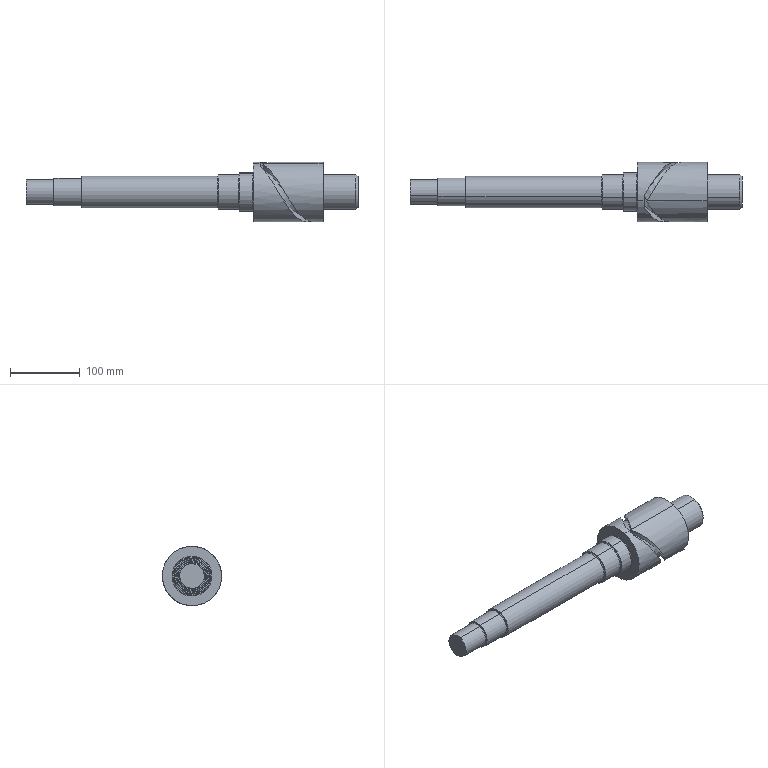Component | SolidWorks | CamAxis-1 | 1 solid | 46 faces | volume 1150566 mm3 | cylinder 16 | torus 10 | plane 10 | spline 8 | cone 2 | commonest cylinder face diameters 50 x4 85 x4 35 x2 40 x2 45 x2 55 x2